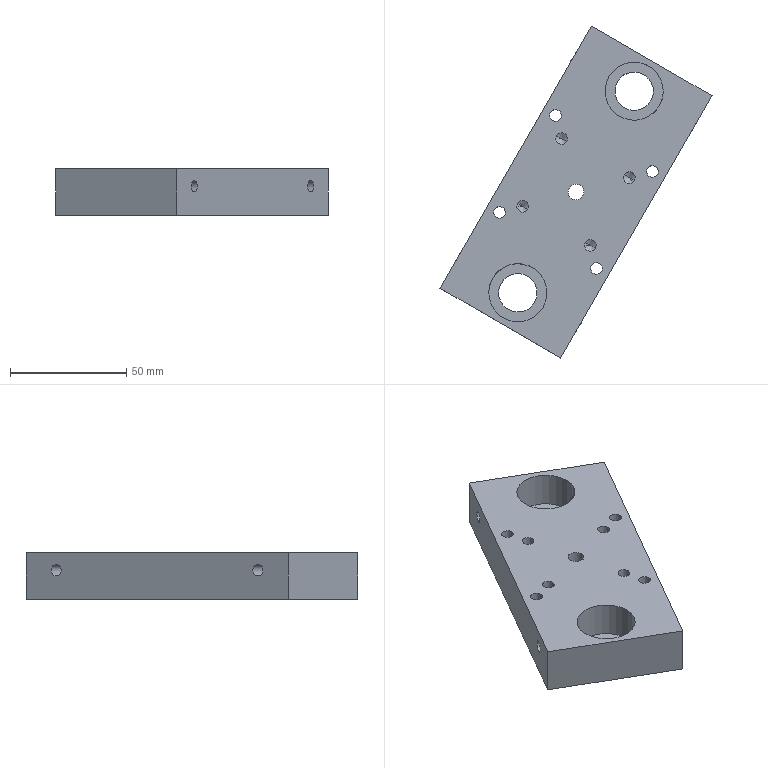Component | SolidWorks | SpindleFixtureAssemblyLeft-1_KLHFH010_38LocatingPinFixingSeat-1 | 1 solid | 53 faces | box 116.96 x 142.58 x 20 mm | volume 126628 mm3 | cylinder 36 | plane 9 | cone 8 | commonest cylinder face diameters 5 x24 16.5 x4 25 x4 6.8 x2 45 x2 | material Plain Carbon Steel
build123d program:
from build123d import *

# Parameters (mm, degrees)
SKETCH1_W           = 60
SKETCH1_H           = 130
BOSS_EXTRUDE1_DEPTH = 10
SKETCH2_R           = 22.5
CUT_EXTRUDE1_DEPTH  = 5
M8_TAPPED_HOLE1_D   = 6.8
SKETCH5_R           = 12.5
CUT_EXTRUDE2_DEPTH  = 15
SKETCH6_R           = 8.25
CUT_EXTRUDE3_DEPTH  = 74.144
M6_TAPPED_HOLE2_D   = 5
CIRPATTERN1_COUNT   = 4
CIRPATTERN2_COUNT   = 4
M6_TAPPED_HOLE3_D   = 5


with BuildPart() as part:
    # Sketch1 → Boss-Extrude1 (new, symmetric)
    with BuildSketch(Plane.XY):
        Rectangle(SKETCH1_W, SKETCH1_H)
    extrude(amount=BOSS_EXTRUDE1_DEPTH, both=True)

    # Sketch2 → Cut-Extrude1 (cut)
    with BuildSketch(Plane.XY.offset(10)):
        Circle(SKETCH2_R)
    extrude(amount=-CUT_EXTRUDE1_DEPTH, mode=Mode.SUBTRACT)

    # M8 Tapped Hole1 (through all)
    with Locations(Plane.XY.offset(5)):
        with Locations((0, 0)):
            Hole(M8_TAPPED_HOLE1_D / 2)

    # Sketch5 → Cut-Extrude2 (cut)
    with BuildSketch(Plane.XY.offset(-10)):
        with Locations((0, 50)):
            Circle(SKETCH5_R)
        with Locations((0, -50)):
            Circle(SKETCH5_R)
    extrude(amount=CUT_EXTRUDE2_DEPTH, mode=Mode.SUBTRACT)

    # Sketch6 → Cut-Extrude3 (cut, through all)
    with BuildSketch(Plane(origin=(0, 0, 5), x_dir=(-1, 0, 0), z_dir=(0, 0, -1))):
        with Locations((0, 50)):
            Circle(SKETCH6_R)
        with Locations((0, -50)):
            Circle(SKETCH6_R)
    extrude(amount=-CUT_EXTRUDE3_DEPTH, mode=Mode.SUBTRACT)

    # M6 Tapped Hole2 (through all)
    with Locations(Plane.XY.offset(10)):
        with Locations((-24.042, 24.042)):
            m6_tapped_hole2 = Hole(M6_TAPPED_HOLE2_D / 2)

    # CirPattern1: M6 Tapped Hole2 ×4 about axis
    cirpattern1_axis = Axis((0, 0, 0), (0, 0, 1))
    for i in range(1, CIRPATTERN1_COUNT):
        add(m6_tapped_hole2.rotate(cirpattern1_axis, i * 360 / CIRPATTERN1_COUNT), mode=Mode.SUBTRACT)

    # Sketch9 → M6 Tapped Hole1 (revolve, cut)
    with BuildSketch(Plane(origin=(16.794, 16.794, -10), x_dir=(0, 1, 0), z_dir=(1, 0, 0))):
        Polygon((0, 0), (0, 14.502), (2.5, 13), (2.5, 0), align=None)
    m6_tapped_hole1 = revolve(axis=Axis((16.794, 16.794, -16.35), (0, 0, 1)), mode=Mode.SUBTRACT)

    # CirPattern2: M6 Tapped Hole1 ×4 about axis
    cirpattern2_axis = Axis((0, 0, 0), (0, 0, 1))
    for i in range(1, CIRPATTERN2_COUNT):
        add(m6_tapped_hole1.rotate(cirpattern2_axis, i * 360 / CIRPATTERN2_COUNT), mode=Mode.SUBTRACT)

    # M6 Tapped Hole3 (through all)
    with Locations(Plane(origin=(30, 0, 0), x_dir=(0, 0, -1), z_dir=(1, 0, 0))):
        with Locations((2.5, 50)):
            m6_tapped_hole3 = Hole(M6_TAPPED_HOLE3_D / 2)

    # Mirror1: M6 Tapped Hole3 across plane
    add(m6_tapped_hole3.mirror(Plane.ZX), mode=Mode.SUBTRACT)


solid = part.part

# Placed as in the assembly
solid = solid.moved(Location((0, 0, -221), (-180, 0, -150)))